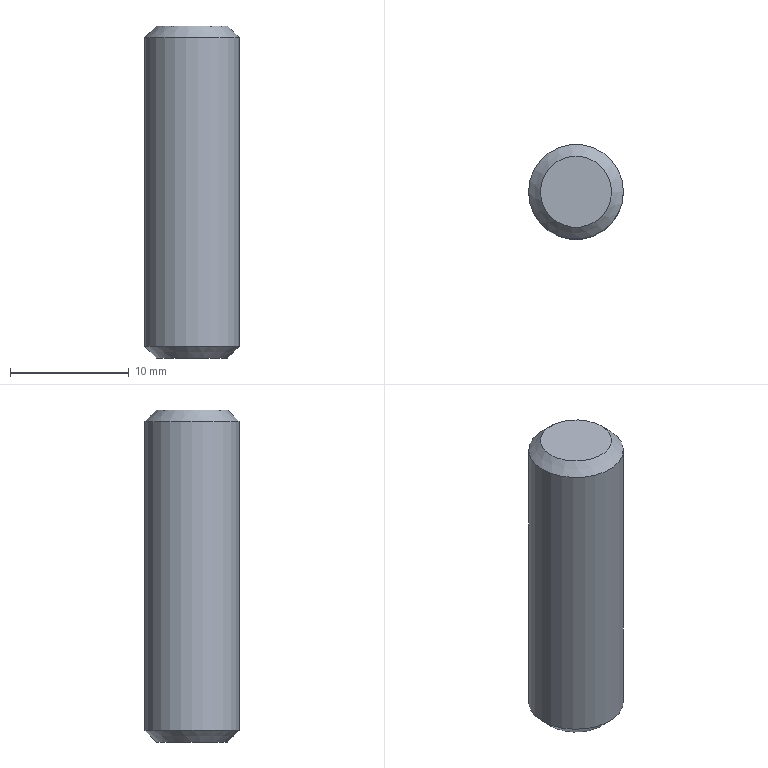Component | NX | PIN | 1 solid | 5 faces | box 8 x 8 x 28 mm | volume 1384 mm3 | plane 2 | cone 2 | cylinder 1 | commonest cylinder face diameters 8 x1
STEP:
#1=CARTESIAN_POINT('',(0.,0.,0.));
#2=DIRECTION('',(0.,0.,1.));
#3=DIRECTION('',(1.,0.,0.));
#4=AXIS2_PLACEMENT_3D('',#1,#2,#3);
#5=CARTESIAN_POINT('',(58.,-0.,-13.));
#6=VERTEX_POINT('',#5);
#7=CARTESIAN_POINT('',(54.,-0.,-13.));
#8=DIRECTION('',(0.,0.,1.));
#9=DIRECTION('',(1.,0.,0.));
#10=AXIS2_PLACEMENT_3D('',#7,#8,#9);
#11=CIRCLE('',#10,4.);
#12=CARTESIAN_POINT('',(54.,-0.,14.));
#13=DIRECTION('',(0.,0.,-1.));
#14=DIRECTION('',(-1.,0.,0.));
#15=AXIS2_PLACEMENT_3D('',#12,#13,#14);
#16=CYLINDRICAL_SURFACE('',#15,4.);
#17=CARTESIAN_POINT('',(9.425,27.));
#18=DIRECTION('',(-1.,0.));
#19=VECTOR('',#18,1.);
#20=LINE('',#17,#19);
#21=(GEOMETRIC_REPRESENTATION_CONTEXT(2)PARAMETRIC_REPRESENTATION_CONTEXT()REPRESENTATION_CONTEXT('',''));
#22=DEFINITIONAL_REPRESENTATION('',(#20),#21);
#23=PCURVE('',#16,#22);
#24=CARTESIAN_POINT('',(54.,-0.,-13.));
#25=DIRECTION('',(0.,0.,1.));
#26=DIRECTION('',(1.,0.,0.));
#27=AXIS2_PLACEMENT_3D('',#24,#25,#26);
#28=CONICAL_SURFACE('',#27,4.,0.7854);
#29=CARTESIAN_POINT('',(0.,0.));
#30=DIRECTION('',(1.,0.));
#31=VECTOR('',#30,1.);
#32=LINE('',#29,#31);
#33=(GEOMETRIC_REPRESENTATION_CONTEXT(2)PARAMETRIC_REPRESENTATION_CONTEXT()REPRESENTATION_CONTEXT('',''));
#34=DEFINITIONAL_REPRESENTATION('',(#32),#33);
#35=PCURVE('',#28,#34);
#36=SURFACE_CURVE('',#11,(#23,#35),.PCURVE_S1.);
#37=EDGE_CURVE('',#6,#6,#36,.T.);
#38=ORIENTED_EDGE('',*,*,#37,.T.);
#39=CARTESIAN_POINT('',(58.,-0.,13.));
#40=VERTEX_POINT('',#39);
#41=CARTESIAN_POINT('',(58.,-0.,13.));
#42=CARTESIAN_POINT('',(58.,-0.,-13.));
#43=B_SPLINE_CURVE_WITH_KNOTS('',1,(#41,#42),.UNSPECIFIED.,.F.,.F.,(2,2),(1.,27.),.PIECEWISE_BEZIER_KNOTS.);
#44=CARTESIAN_POINT('',(3.142,0.));
#45=DIRECTION('',(0.,1.));
#46=VECTOR('',#45,1.);
#47=LINE('',#44,#46);
#48=(GEOMETRIC_REPRESENTATION_CONTEXT(2)PARAMETRIC_REPRESENTATION_CONTEXT()REPRESENTATION_CONTEXT('',''));
#49=DEFINITIONAL_REPRESENTATION('',(#47),#48);
#50=PCURVE('',#16,#49);
#51=CARTESIAN_POINT('',(9.425,0.));
#52=DIRECTION('',(0.,1.));
#53=VECTOR('',#52,1.);
#54=LINE('',#51,#53);
#55=(GEOMETRIC_REPRESENTATION_CONTEXT(2)PARAMETRIC_REPRESENTATION_CONTEXT()REPRESENTATION_CONTEXT('',''));
#56=DEFINITIONAL_REPRESENTATION('',(#54),#55);
#57=PCURVE('',#16,#56);
#58=SEAM_CURVE('',#43,(#50,#57),.PCURVE_S1.);
#59=EDGE_CURVE('',#40,#6,#58,.T.);
#60=ORIENTED_EDGE('',*,*,#59,.F.);
#61=CARTESIAN_POINT('',(54.,-0.,13.));
#62=DIRECTION('',(0.,0.,-1.));
#63=DIRECTION('',(1.,0.,0.));
#64=AXIS2_PLACEMENT_3D('',#61,#62,#63);
#65=CIRCLE('',#64,4.);
#66=CARTESIAN_POINT('',(3.142,1.));
#67=DIRECTION('',(1.,0.));
#68=VECTOR('',#67,1.);
#69=LINE('',#66,#68);
#70=(GEOMETRIC_REPRESENTATION_CONTEXT(2)PARAMETRIC_REPRESENTATION_CONTEXT()REPRESENTATION_CONTEXT('',''));
#71=DEFINITIONAL_REPRESENTATION('',(#69),#70);
#72=PCURVE('',#16,#71);
#73=CARTESIAN_POINT('',(54.,-0.,14.));
#74=DIRECTION('',(0.,0.,-1.));
#75=DIRECTION('',(-1.,0.,0.));
#76=AXIS2_PLACEMENT_3D('',#73,#74,#75);
#77=CONICAL_SURFACE('',#76,3.,0.7854);
#78=CARTESIAN_POINT('',(3.142,1.));
#79=DIRECTION('',(1.,0.));
#80=VECTOR('',#79,1.);
#81=LINE('',#78,#80);
#82=(GEOMETRIC_REPRESENTATION_CONTEXT(2)PARAMETRIC_REPRESENTATION_CONTEXT()REPRESENTATION_CONTEXT('',''));
#83=DEFINITIONAL_REPRESENTATION('',(#81),#82);
#84=PCURVE('',#77,#83);
#85=SURFACE_CURVE('',#65,(#72,#84),.PCURVE_S1.);
#86=EDGE_CURVE('',#40,#40,#85,.T.);
#87=ORIENTED_EDGE('',*,*,#86,.T.);
#88=ORIENTED_EDGE('',*,*,#59,.T.);
#89=EDGE_LOOP('',(#38,#60,#87,#88));
#90=FACE_BOUND('',#89,.T.);
#91=ADVANCED_FACE('',(#90),#16,.T.);
#92=CARTESIAN_POINT('',(57.,-0.,14.));
#93=VERTEX_POINT('',#92);
#94=CARTESIAN_POINT('',(54.,-0.,14.));
#95=DIRECTION('',(0.,0.,1.));
#96=DIRECTION('',(1.,0.,0.));
#97=AXIS2_PLACEMENT_3D('',#94,#95,#96);
#98=CIRCLE('',#97,3.);
#99=CARTESIAN_POINT('',(54.,-0.,14.));
#100=DIRECTION('',(0.,0.,1.));
#101=DIRECTION('',(1.,0.,0.));
#102=AXIS2_PLACEMENT_3D('',#99,#100,#101);
#103=PLANE('',#102);
#104=CARTESIAN_POINT('',(0.,0.));
#105=DIRECTION('',(1.,0.));
#106=AXIS2_PLACEMENT_2D('',#104,#105);
#107=CIRCLE('',#106,3.);
#108=(GEOMETRIC_REPRESENTATION_CONTEXT(2)PARAMETRIC_REPRESENTATION_CONTEXT()REPRESENTATION_CONTEXT('',''));
#109=DEFINITIONAL_REPRESENTATION('',(#107),#108);
#110=PCURVE('',#103,#109);
#111=CARTESIAN_POINT('',(9.425,0.));
#112=DIRECTION('',(-1.,0.));
#113=VECTOR('',#112,1.);
#114=LINE('',#111,#113);
#115=(GEOMETRIC_REPRESENTATION_CONTEXT(2)PARAMETRIC_REPRESENTATION_CONTEXT()REPRESENTATION_CONTEXT('',''));
#116=DEFINITIONAL_REPRESENTATION('',(#114),#115);
#117=PCURVE('',#77,#116);
#118=SURFACE_CURVE('',#98,(#110,#117),.PCURVE_S1.);
#119=EDGE_CURVE('',#93,#93,#118,.T.);
#120=ORIENTED_EDGE('',*,*,#119,.T.);
#121=EDGE_LOOP('',(#120));
#122=FACE_BOUND('',#121,.T.);
#123=ADVANCED_FACE('',(#122),#103,.T.);
#124=CARTESIAN_POINT('',(57.,-0.,-14.));
#125=VERTEX_POINT('',#124);
#126=CARTESIAN_POINT('',(54.,-0.,-14.));
#127=DIRECTION('',(0.,0.,-1.));
#128=DIRECTION('',(1.,0.,0.));
#129=AXIS2_PLACEMENT_3D('',#126,#127,#128);
#130=CIRCLE('',#129,3.);
#131=CARTESIAN_POINT('',(54.,-0.,-14.));
#132=DIRECTION('',(0.,0.,1.));
#133=DIRECTION('',(1.,0.,0.));
#134=AXIS2_PLACEMENT_3D('',#131,#132,#133);
#135=PLANE('',#134);
#136=CARTESIAN_POINT('',(3.,0.));
#137=CARTESIAN_POINT('',(3.,-5.196));
#138=CARTESIAN_POINT('',(-1.5,-2.598));
#139=CARTESIAN_POINT('',(-6.,-0.));
#140=CARTESIAN_POINT('',(-1.5,2.598));
#141=CARTESIAN_POINT('',(3.,5.196));
#142=CARTESIAN_POINT('',(3.,0.));
#143=(BOUNDED_CURVE()B_SPLINE_CURVE(2,(#136,#137,#138,#139,#140,#141,#142),.UNSPECIFIED.,.T.,.F.)B_SPLINE_CURVE_WITH_KNOTS((1,2,2,2,2,1),(-2.094,0.,2.094,4.189,6.283,8.378),.UNSPECIFIED.)CURVE()GEOMETRIC_REPRESENTATION_ITEM()RATIONAL_B_SPLINE_CURVE((1.,0.5,1.,0.5,1.,0.5,1.))REPRESENTATION_ITEM(''));
#144=(GEOMETRIC_REPRESENTATION_CONTEXT(2)PARAMETRIC_REPRESENTATION_CONTEXT()REPRESENTATION_CONTEXT('',''));
#145=DEFINITIONAL_REPRESENTATION('',(#143),#144);
#146=PCURVE('',#135,#145);
#147=CARTESIAN_POINT('',(6.283,-1.));
#148=DIRECTION('',(-1.,0.));
#149=VECTOR('',#148,1.);
#150=LINE('',#147,#149);
#151=(GEOMETRIC_REPRESENTATION_CONTEXT(2)PARAMETRIC_REPRESENTATION_CONTEXT()REPRESENTATION_CONTEXT('',''));
#152=DEFINITIONAL_REPRESENTATION('',(#150),#151);
#153=PCURVE('',#28,#152);
#154=SURFACE_CURVE('',#130,(#146,#153),.PCURVE_S1.);
#155=EDGE_CURVE('',#125,#125,#154,.T.);
#156=ORIENTED_EDGE('',*,*,#155,.T.);
#157=EDGE_LOOP('',(#156));
#158=FACE_BOUND('',#157,.T.);
#159=ADVANCED_FACE('',(#158),#135,.F.);
#160=ORIENTED_EDGE('',*,*,#155,.F.);
#161=CARTESIAN_POINT('',(57.,-0.,-14.));
#162=CARTESIAN_POINT('',(58.,-0.,-13.));
#163=B_SPLINE_CURVE_WITH_KNOTS('',1,(#161,#162),.UNSPECIFIED.,.F.,.F.,(2,2),(-1.414,0.),.PIECEWISE_BEZIER_KNOTS.);
#164=CARTESIAN_POINT('',(6.283,0.));
#165=DIRECTION('',(0.,1.));
#166=VECTOR('',#165,1.);
#167=LINE('',#164,#166);
#168=(GEOMETRIC_REPRESENTATION_CONTEXT(2)PARAMETRIC_REPRESENTATION_CONTEXT()REPRESENTATION_CONTEXT('',''));
#169=DEFINITIONAL_REPRESENTATION('',(#167),#168);
#170=PCURVE('',#28,#169);
#171=CARTESIAN_POINT('',(0.,0.));
#172=DIRECTION('',(0.,1.));
#173=VECTOR('',#172,1.);
#174=LINE('',#171,#173);
#175=(GEOMETRIC_REPRESENTATION_CONTEXT(2)PARAMETRIC_REPRESENTATION_CONTEXT()REPRESENTATION_CONTEXT('',''));
#176=DEFINITIONAL_REPRESENTATION('',(#174),#175);
#177=PCURVE('',#28,#176);
#178=SEAM_CURVE('',#163,(#170,#177),.PCURVE_S1.);
#179=EDGE_CURVE('',#125,#6,#178,.T.);
#180=ORIENTED_EDGE('',*,*,#179,.T.);
#181=ORIENTED_EDGE('',*,*,#37,.F.);
#182=ORIENTED_EDGE('',*,*,#179,.F.);
#183=EDGE_LOOP('',(#160,#180,#181,#182));
#184=FACE_BOUND('',#183,.T.);
#185=ADVANCED_FACE('',(#184),#28,.T.);
#186=ORIENTED_EDGE('',*,*,#86,.F.);
#187=CARTESIAN_POINT('',(57.,-0.,14.));
#188=CARTESIAN_POINT('',(58.,-0.,13.));
#189=B_SPLINE_CURVE_WITH_KNOTS('',1,(#187,#188),.UNSPECIFIED.,.F.,.F.,(2,2),(0.,1.414),.PIECEWISE_BEZIER_KNOTS.);
#190=CARTESIAN_POINT('',(3.142,0.));
#191=DIRECTION('',(0.,1.));
#192=VECTOR('',#191,1.);
#193=LINE('',#190,#192);
#194=(GEOMETRIC_REPRESENTATION_CONTEXT(2)PARAMETRIC_REPRESENTATION_CONTEXT()REPRESENTATION_CONTEXT('',''));
#195=DEFINITIONAL_REPRESENTATION('',(#193),#194);
#196=PCURVE('',#77,#195);
#197=CARTESIAN_POINT('',(9.425,0.));
#198=DIRECTION('',(0.,1.));
#199=VECTOR('',#198,1.);
#200=LINE('',#197,#199);
#201=(GEOMETRIC_REPRESENTATION_CONTEXT(2)PARAMETRIC_REPRESENTATION_CONTEXT()REPRESENTATION_CONTEXT('',''));
#202=DEFINITIONAL_REPRESENTATION('',(#200),#201);
#203=PCURVE('',#77,#202);
#204=SEAM_CURVE('',#189,(#196,#203),.PCURVE_S1.);
#205=EDGE_CURVE('',#93,#40,#204,.T.);
#206=ORIENTED_EDGE('',*,*,#205,.F.);
#207=ORIENTED_EDGE('',*,*,#119,.F.);
#208=ORIENTED_EDGE('',*,*,#205,.T.);
#209=EDGE_LOOP('',(#186,#206,#207,#208));
#210=FACE_BOUND('',#209,.T.);
#211=ADVANCED_FACE('',(#210),#77,.T.);
#212=CLOSED_SHELL('',(#91,#123,#159,#185,#211));
#213=MANIFOLD_SOLID_BREP('',#212);
#214=(LENGTH_UNIT()NAMED_UNIT(*)SI_UNIT(.MILLI.,.METRE.));
#215=UNCERTAINTY_MEASURE_WITH_UNIT(LENGTH_MEASURE(0.00001),#214,'','');
#216=(NAMED_UNIT(*)PLANE_ANGLE_UNIT()SI_UNIT($,.RADIAN.));
#217=(NAMED_UNIT(*)SI_UNIT($,.STERADIAN.)SOLID_ANGLE_UNIT());
#218=(GEOMETRIC_REPRESENTATION_CONTEXT(3)GLOBAL_UNCERTAINTY_ASSIGNED_CONTEXT((#215))GLOBAL_UNIT_ASSIGNED_CONTEXT((#214,#216,#217))REPRESENTATION_CONTEXT('',''));
#219=ADVANCED_BREP_SHAPE_REPRESENTATION('',(#4,#213),#218);